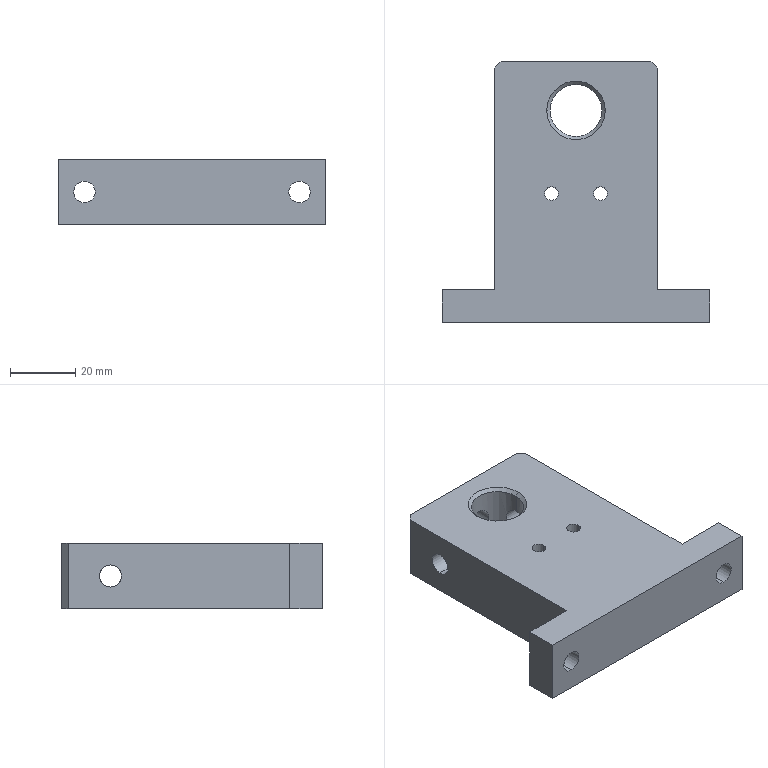Component | SolidWorks | SL010-LeftStreamline-1-1_SL010-2M-0112-000-2-1-1_SL010-LXFB-0102010-1-1 | 1 solid | 35 faces | box 82 x 80 x 20 mm | volume 79383 mm3 | cylinder 16 | plane 15 | cone 4 | commonest cylinder face diameters 6.8 x6 4.2 x4 6.6 x4 16 x2 | material S45C
build123d program:
from build123d import *

# Parameters (mm, degrees)
SKETCH1_2_W            = 50
SKETCH1_2_H            = 80
BOSS_EXTRUDE1_DEPTH    = 10
M16_TAPPED_HOLE1_D     = 16
M16_TAPPED_HOLE1_DEPTH = 38
M16_TAPPED_HOLE1_TIP   = 4.807
CHAMFER2_SIZE          = 1
SKETCH4_W              = 82
SKETCH4_H              = 20
BOSS_EXTRUDE2_DEPTH    = 10
SKETCH5_R              = 3.3
CUT_EXTRUDE1_2_DEPTH   = 82.737
M8_TAPPED_HOLE1_D      = 6.8
M8_TAPPED_HOLE1_DEPTH  = 19.75
M8_TAPPED_HOLE1_TIP    = 2.043
M5_TAPPED_HOLE1_D      = 4.2
CHAMFER1_SIZE          = 2
M8_TAPPED_HOLE2_D      = 6.8
SKETCH1_W              = 8
SKETCH1_H              = 9.6
CUT_EXTRUDE1_DEPTH     = 2


with BuildPart() as part:
    # Sketch1_2 → Boss-Extrude1 (new, symmetric)
    with BuildSketch(Plane.XY):
        Rectangle(SKETCH1_2_W, SKETCH1_2_H)
    extrude(amount=BOSS_EXTRUDE1_DEPTH, both=True)

    # M16 Tapped Hole1
    with Locations(Plane.XY.offset(10)):
        with Locations((0, 25)):
            Hole(M16_TAPPED_HOLE1_D / 2, depth=M16_TAPPED_HOLE1_DEPTH)
            with Locations((0, 0, -(M16_TAPPED_HOLE1_DEPTH + M16_TAPPED_HOLE1_TIP / 2))):  # 118° drill point
                Cone(0, M16_TAPPED_HOLE1_D / 2, M16_TAPPED_HOLE1_TIP, mode=Mode.SUBTRACT)

    # Chamfer2
    chamfer2_edges = [part.edges().sort_by_distance(p)[0] for p in [
        (8, 25, -10),
        (8, 25, 10),
    ]]
    chamfer(chamfer2_edges, length=CHAMFER2_SIZE)

    # Sketch4 → Boss-Extrude2 (add)
    with BuildSketch(Plane.XZ.offset(40)):
        Rectangle(SKETCH4_W, SKETCH4_H)
    extrude(amount=-BOSS_EXTRUDE2_DEPTH)

    # Sketch5 → Cut-Extrude1_2 (cut, through all)
    with BuildSketch(Plane(origin=(0, -30, 0), x_dir=(1, 0, 0), z_dir=(0, 1, 0))):
        with Locations(Location((33, 0, 0), (0, 0, 270))):
            Circle(SKETCH5_R)
        with Locations(Location((-33, 0, 0), (0, 0, 270))):
            Circle(SKETCH5_R)
    extrude(amount=-CUT_EXTRUDE1_2_DEPTH, mode=Mode.SUBTRACT)

    # M8 Tapped Hole1
    with Locations(Plane(origin=(0, 40, 0), x_dir=(1, 0, 0), z_dir=(0, 1, 0))):
        with Locations((0, 0)):
            Hole(M8_TAPPED_HOLE1_D / 2, depth=M8_TAPPED_HOLE1_DEPTH)
            with Locations((0, 0, -(M8_TAPPED_HOLE1_DEPTH + M8_TAPPED_HOLE1_TIP / 2))):  # 118° drill point
                Cone(0, M8_TAPPED_HOLE1_D / 2, M8_TAPPED_HOLE1_TIP, mode=Mode.SUBTRACT)

    # M5 Tapped Hole1 (through all)
    with Locations(Plane(origin=(0, 0, -10), x_dir=(-1, 0, 0), z_dir=(0, 0, -1))):
        with Locations((7.5, -0.5), (-7.5, -0.5)):
            Hole(M5_TAPPED_HOLE1_D / 2)

    # Chamfer1
    chamfer1_edges = [part.edges().sort_by_distance(p)[0] for p in [
        (-25, 40, 0),
        (25, 40, 0),
    ]]
    chamfer(chamfer1_edges, length=CHAMFER1_SIZE)

    # M8 Tapped Hole2 (through all)
    with Locations(Plane(origin=(25, 0, 0), x_dir=(0, 0, -1), z_dir=(1, 0, 0))):
        with Locations((0, 25)):
            Hole(M8_TAPPED_HOLE2_D / 2)

    # Sketch1 → Cut-Extrude1 (cut)
    with BuildSketch(Plane(origin=(0, 0, -10), x_dir=(-1, 0, 0), z_dir=(0, 0, -1))):
        with Locations((-22, 36.204)):
            Rectangle(SKETCH1_W, SKETCH1_H)
    extrude(amount=-CUT_EXTRUDE1_DEPTH, mode=Mode.SUBTRACT)


solid = part.part

# Placed as in the assembly
solid = solid.moved(Location((-175, -189.904, -703.035), (0, 0, 0)))